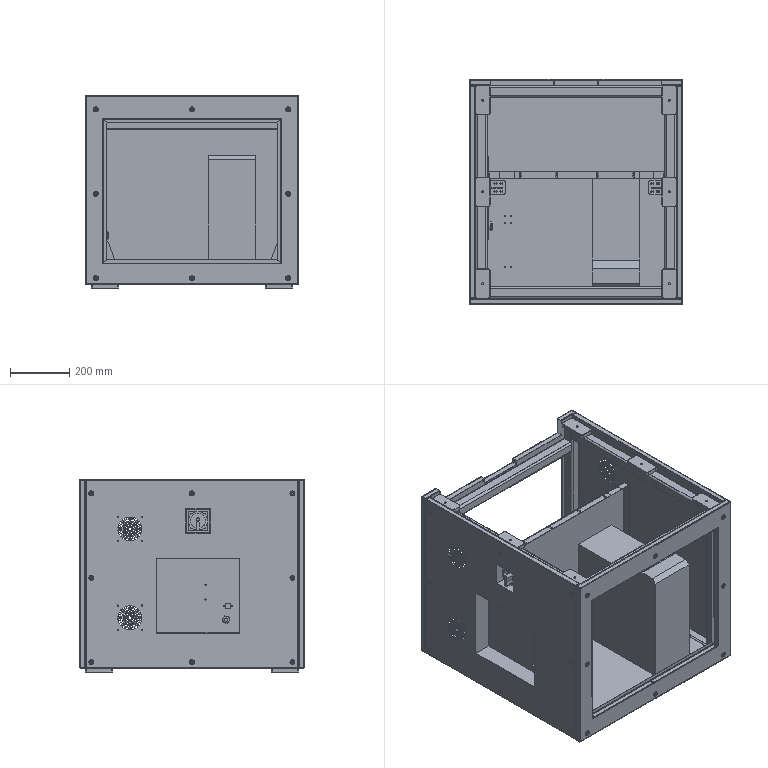Assembly | SolidWorks | mm | 22 component files | 35 solids | 2904 faces | box 720 x 760 x 652 mm | volume 31247087 mm3 | cylinder 1368 | plane 937 | torus 267 | spline 220 | cone 112 | commonest cylinder face diameters 5 x412 6.5 x86 15 x62 12 x62 6 x60 14 x48 1.473 x47 6.8 x44
Bill of materials:
01FrameBody | 1 | 4040 Square Tube | Open rectangular box-shaped frame made of square-section members: four vertical corner posts joined by horizontal rails at top and bottom on all four sides.
02LowerRackSpacer | 6 | A3 Steel | Rectangular block or thick plate with rounded corners, chamfered top and bottom edges, and one round through-hole in the centre.
03IntegratedCasterMount | 4 | A3 Steel | Square thick plate with small chamfered corners, chamfered edges, and four through-holes near the corners.
04CounterweightPlate | 1 | A3 Steel | Thin flat square sheet with slightly cut corners and a scattered pattern of small holes, some in four-hole groups and some single.
01-06LeftGuardPlate | 1 | SPCC | Flat rectangular panel with two round vent patterns, each made of concentric arc slots with a central hole and four small holes around it, plus eight holes spaced around the edge.
01-07RightGuardPlate | 1 | SPCC | Rectangular panel similar to a perforated plate, with two round slotted vent patterns, eight edge holes, and two raised rectangular box-shaped blocks on one face. It also has a small square cutout, a round hole and several small holes.
01-10ElectricalControlPanel | 1 | SGLCC | Shallow rectangular tray or pan: a flat panel with folded-up edges on all four sides. The longer flanges have elongated slots and the shorter flanges have round holes.
01-11FrontGuardPlate | 1 | SPCC | Flat rectangular frame with a large rectangular window that has a bevelled or stepped inner edge. The top edge has a tab rising at each end and a shallow notch in the middle. There are seven holes around the frame.
01-12RearGuardPlate | 1 | SPCC | Flat rectangular frame with a large rectangular window that has a bevelled or recessed inner edge, and eight holes evenly placed around the border.
01-16ElectricalControlPanelBracket | 1 | SGLCC | L-shaped bracket: a tall tapered vertical plate with three holes along one edge, a horizontal base flange with four elongated slots and rounded corners, and a triangular gusset between the two.
CableGlandPG13.5Black | 1 |  | Round hollow fitting with a domed end, a hexagonal nut section, a grooved neck, a larger hexagonal collar, and a grooved or ridged tube end. A round bore runs all the way through.
Host | 1 | Domestic 6061 | Solid rectangular block with a stepped, chamfered raised strip at one end of its top face, so one side profile has a small raised lip with angled edges.
Mirror01-16ElectricalControlPanelBracket | 1 | SUS304 | L-shaped plate bracket: a tall vertical web with one straight edge and one tapered edge, joined at a right angle to a short base flange that has four slotted holes. A triangular gusset plate runs between the flange and the web.
PowerSwitchTDS25-FRR | 1 |  | Flanged cylindrical body: a square plate with rounded corners and four corner holes, a short cylindrical shaft sticking out from the front face, a larger round disc-shaped body behind the plate, and a further protrusion on the rear.
Mates:
1. coincident | 01-01FrameBody-1/03IntegratedCasterMount-1 face at (0, 0, 0) dir (0, 0, -1) | assembly plane at (0, 0, 0) dir (0, 0, 1)
2. coincident | 01-01FrameBody-1/03IntegratedCasterMount-1 face at (-92, 0, 0) dir (0, -1, 0) | assembly plane at (0, 0, 0) dir (0, 1, 0)
3. coincident | 01-01FrameBody-1/03IntegratedCasterMount-1 face at (0, 92, 0) dir (1, 0, 0) | assembly plane at (0, 0, 0) dir (1, 0, 0)
4. coincident | 01-01FrameBody-1/01FrameBody-2 face at (-7, 720, 35) dir (0, 1, 0) | 01-11FrontGuardPlate-1 face at (6, 720, 17.207) dir (0, -1, 0)
5. coincident | 01-01FrameBody-1/01FrameBody-2 face at (-20, 687, 15) dir (0, 0, -1) | 01-11FrontGuardPlate-1 face at (-700, 720, 15) dir (0, 0, -1)
6. width | 01-11FrontGuardPlate-1 face at (20, 720, 15) dir (1, 0, 0) | 01-11FrontGuardPlate-1 face at (-700, 738.5, 15) dir (-1, 0, 0) | 01-01FrameBody-1/01FrameBody-2 face at (-680, 687, 35) dir (-1, 0, 0) | 01-01FrameBody-1/01FrameBody-2 face at (0, 687, 35) dir (1, 0, 0)
7. coincident | 01-01FrameBody-1/01FrameBody-2 face at (-20, 0, 618) dir (0, -1, 0) | 01-12RearGuardPlate-1 face at (17.793, 0, 650.5) dir (0, 1, 0)
8. coincident | 01-11FrontGuardPlate-1 face at (-700, 738.5, 15) dir (-1, 0, 0) | 01-12RearGuardPlate-1 face at (-700, 0, 15) dir (-1, 0, 0)
9. coincident | 01-11FrontGuardPlate-1 face at (20, 720, 652) dir (0, 0, 1) | 01-12RearGuardPlate-1 face at (-700, 0, 652) dir (0, 0, 1)
10. coincident | 01-01FrameBody-1/01FrameBody-2 face at (0, 20, 592) dir (1, 0, 0) | 01-06LeftGuardPlate-1 face at (0, 2.707, 638) dir (-1, 0, 0)
11. width | 01-06LeftGuardPlate-1 face at (0, 0.5, 15) dir (0, -1, 0) | 01-06LeftGuardPlate-1 face at (18.5, 719.5, 15) dir (0, 1, 0) | 01-11FrontGuardPlate-1 face at (20, 740, 652) dir (0, 1, 0) | 01-12RearGuardPlate-1 face at (-700, -20, 652) dir (0, -1, 0)
12. coincident | 01-06LeftGuardPlate-1 face at (0, 0.5, 652) dir (0, 0, 1) | 01-12RearGuardPlate-1 face at (-700, 0, 652) dir (0, 0, 1)
13. coincident | 01-01FrameBody-1/01FrameBody-2 face at (-680, 20, 592) dir (-1, 0, 0) | 01-07RightGuardPlate-1 face at (-680, 717.293, 638) dir (1, 0, 0)
14. coincident | 01-07RightGuardPlate-1 face at (-680, 719.5, 652) dir (0, 0, 1) | 01-12RearGuardPlate-1 face at (-700, 0, 652) dir (0, 0, 1)
15. width | 01-07RightGuardPlate-1 face at (-680, 719.5, 15) dir (0, 1, 0) | 01-07RightGuardPlate-1 face at (-698.5, 0.5, 15) dir (0, -1, 0) | 01-12RearGuardPlate-1 face at (-700, -20, 652) dir (0, -1, 0) | 01-11FrontGuardPlate-1 face at (20, 740, 652) dir (0, 1, 0)
16. coincident | 01-01FrameBody-1/04CounterweightPlate-4 face at (-640, 680, 55) dir (0, 0, 1) | 01-10ElectricalControlPanel-1 face at (-632, 405, 55) dir (0, 0, -1)
17. distance | 01-01FrameBody-1/01FrameBody-2 face at (0, 20, 22) dir (1, 0, 0) | 01-10ElectricalControlPanel-1 face at (-40, 405, 57) dir (1, 0, 0)
18. distance | 01-10ElectricalControlPanel-1 face at (-632, 430, 57) dir (0, 1, 0) | 01-01FrameBody-1/01FrameBody-2 face at (-20, 680, 48) dir (0, -1, 0)
19. coincident | 01-01FrameBody-1/04CounterweightPlate-4 face at (-640, 680, 55) dir (0, 0, 1) | Host-1 face at (-124.631, 35, 55) dir (0, 0, -1)
20. coincident | 01-01FrameBody-1/04CounterweightPlate-4 face at (-640, 680, 55) dir (0, 0, 1) | 01-16ElectricalControlPanelBracket-1 face at (-629, 353, 55) dir (0, 0, -1)
21. coincident | 01-10ElectricalControlPanel-1 face at (-632, 405, 537) dir (1, 0, 0) | 01-16ElectricalControlPanelBracket-1 face at (-632, 353, 258) dir (-1, 0, 0)
22. distance | 01-10ElectricalControlPanel-1 face at (-632, 428, 57) dir (0, -1, 0) | 01-16ElectricalControlPanelBracket-1 face at (-628.263, 418, 55) dir (0, 1, 0)
23. coincident | 01-10ElectricalControlPanel-1 face at (-632, 405, 55) dir (0, -1, 0) | Host-1 face at (-284.631, 405, 415) dir (0, 1, 0)
24. coincident | 01-07RightGuardPlate-1 face at (-660, 360, 333.5) dir (-1, 0, 0) | PowerSwitchTDS25-FRR-1 face at (-660, 372, 479.5) dir (1, 0, 0)
25. width | 01-07RightGuardPlate-1 face at (-658.5, 299.5, 333.5) dir (0, 1, 0) | 01-07RightGuardPlate-1 face at (-658.5, 379.5, 333.5) dir (0, -1, 0) | PowerSwitchTDS25-FRR-1 face at (-667, 307, 544.5) dir (0, -1, 0) | PowerSwitchTDS25-FRR-1 face at (-667, 372, 544.5) dir (0, 1, 0)
26. width | 01-07RightGuardPlate-1 face at (-658.5, 360, 552) dir (0, 0, -1) | 01-07RightGuardPlate-1 face at (-658.5, 360, 472) dir (0, 0, 1) | PowerSwitchTDS25-FRR-1 face at (-667, 372, 544.5) dir (0, 0, 1) | PowerSwitchTDS25-FRR-1 face at (-667, 372, 479.5) dir (0, 0, -1)
27. coincident | 01-07RightGuardPlate-1 face at (-638.5, 480, 383.5) dir (-1, 0, 0) | CableGlandPG13.5Black-1 face at (-638.5, 258.069, 180.851) dir (1, 0, 0)
28. concentric | 01-07RightGuardPlate-1 face at (-637, 245, 178.5) dir (-1, 0, 0) r 11.25 | CableGlandPG13.5Black-1 face at (-621.473, 245, 178.5) dir (-1, 0, 0) r 5.5
29. coincident | 03IntegratedCasterMount-2 face at (260.665, -242.877, -292.639) dir (0, 0, 1) | 01FrameBody-2 face at (260.665, -314.877, -292.639) dir (0, 0, -1)
30. coincident | 01FrameBody-2 face at (260.665, -327.877, -272.639) dir (1, 0, 0) | 03IntegratedCasterMount-2 face at (260.665, -334.877, -307.639) dir (1, 0, 0)
31. coincident | 01FrameBody-2 face at (227.665, -334.877, -272.639) dir (0, -1, 0) | 03IntegratedCasterMount-2 face at (168.665, -334.877, -307.639) dir (0, -1, 0)
32. coincident | 01FrameBody-2 face at (220.665, 325.123, -292.639) dir (0, 0, -1) | 03IntegratedCasterMount-3 face at (260.665, 345.123, -292.639) dir (0, 0, 1)
33. coincident | 01FrameBody-2 face at (227.665, 345.123, -272.639) dir (0, 1, 0) | 03IntegratedCasterMount-3 face at (168.665, 345.123, -307.639) dir (0, 1, 0)
34. coincident | 01FrameBody-2 face at (260.665, 312.123, -272.639) dir (1, 0, 0) | 03IntegratedCasterMount-3 face at (260.665, 253.123, -307.639) dir (1, 0, 0)
35. coincident | 01FrameBody-2 face at (-459.335, 325.123, -292.639) dir (0, 0, -1) | 03IntegratedCasterMount-4 face at (-367.335, 345.123, -292.639) dir (0, 0, 1)
36. coincident | 01FrameBody-2 face at (-452.335, 345.123, -272.639) dir (0, 1, 0) | 03IntegratedCasterMount-4 face at (-459.335, 345.123, -307.639) dir (0, 1, 0)
37. coincident | 01FrameBody-2 face at (-459.335, 312.123, -272.639) dir (-1, 0, 0) | 03IntegratedCasterMount-4 face at (-459.335, 253.123, -307.639) dir (-1, 0, 0)
38. coincident | 01FrameBody-2 face at (-419.335, -314.877, -292.639) dir (0, 0, -1) | 03IntegratedCasterMount-1 face at (-459.335, -334.877, -292.639) dir (0, 0, 1)
39. coincident | 01FrameBody-2 face at (-459.335, -327.877, -272.639) dir (-1, 0, 0) | 03IntegratedCasterMount-1 face at (-459.335, -242.877, -307.639) dir (-1, 0, 0)
40. coincident | 01FrameBody-2 face at (-452.335, -334.877, -272.639) dir (0, -1, 0) | 03IntegratedCasterMount-1 face at (-367.335, -334.877, -307.639) dir (0, -1, 0)
41. coincident | 01FrameBody-2 face at (-459.335, -314.877, 317.361) dir (0, 0, 1) | 02LowerRackSpacer-1 face at (-359.335, -334.877, 317.361) dir (0, 0, -1)
42. coincident | 01FrameBody-2 face at (-419.335, 325.123, 317.361) dir (0, 0, 1) | 02LowerRackSpacer-2 face at (-359.335, 345.123, 317.361) dir (0, 0, -1)
43. coincident | 01FrameBody-2 face at (240.665, 305.123, 317.361) dir (0, 0, 1) | 02LowerRackSpacer-6 face at (260.665, 295.123, 317.361) dir (0, 0, -1)
44. coincident | 01FrameBody-2 face at (260.665, 312.123, -272.639) dir (1, 0, 0) | 02LowerRackSpacer-6 face at (260.665, 345.123, 317.361) dir (1, 0, 0)
45. coincident | 01FrameBody-2 face at (227.665, 345.123, -272.639) dir (0, 1, 0) | 02LowerRackSpacer-6 face at (160.665, 345.123, 317.361) dir (0, 1, 0)
46. coincident | 01FrameBody-2 face at (240.665, -334.877, 317.361) dir (0, 0, 1) | 02LowerRackSpacer-5 face at (260.665, -334.877, 317.361) dir (0, 0, -1)
47. coincident | 01FrameBody-2 face at (227.665, -334.877, -272.639) dir (0, -1, 0) | 02LowerRackSpacer-5 face at (160.665, -334.877, 317.361) dir (0, -1, 0)
48. coincident | 01FrameBody-2 face at (260.665, -327.877, -272.639) dir (1, 0, 0) | 02LowerRackSpacer-5 face at (260.665, -284.877, 317.361) dir (1, 0, 0)
49. coincident | 01FrameBody-2 face at (-459.335, -327.877, -272.639) dir (-1, 0, 0) | 02LowerRackSpacer-1 face at (-459.335, -284.877, 317.361) dir (-1, 0, 0)
50. coincident | 01FrameBody-2 face at (-452.335, -334.877, -272.639) dir (0, -1, 0) | 02LowerRackSpacer-1 face at (-459.335, -334.877, 317.361) dir (0, -1, 0)
51. coincident | 01FrameBody-2 face at (-459.335, 312.123, -272.639) dir (-1, 0, 0) | 02LowerRackSpacer-2 face at (-459.335, 295.123, 332.361) dir (-1, 0, 0)
52. coincident | 01FrameBody-2 face at (-452.335, 345.123, -272.639) dir (0, 1, 0) | 02LowerRackSpacer-2 face at (-459.335, 345.123, 332.361) dir (0, 1, 0)
53. width | 04CounterweightPlate-4 face at (-419.335, -294.877, -252.639) dir (-1, 0, 0) | 04CounterweightPlate-4 face at (220.665, -294.877, -252.639) dir (1, 0, 0) | 01FrameBody-2 face at (260.665, -314.877, -259.639) dir (1, 0, 0) | 01FrameBody-2 face at (-459.335, -314.877, -259.639) dir (-1, 0, 0)
54. width | 04CounterweightPlate-4 face at (-419.335, -294.877, -252.639) dir (0, -1, 0) | 04CounterweightPlate-4 face at (-419.335, 305.123, -252.639) dir (0, 1, 0) | 01FrameBody-2 face at (-439.335, 345.123, -285.639) dir (0, 1, 0) | 01FrameBody-2 face at (-439.335, -334.877, -285.639) dir (0, -1, 0)
55. coincident | 01FrameBody-2 face at (-439.335, 338.123, -252.639) dir (0, 0, 1) | 04CounterweightPlate-4 face at (220.665, 305.123, -252.639) dir (0, 0, 1)
56. coincident | 01FrameBody-2 face at (-439.335, -301.877, 317.361) dir (0, 0, 1) | 02LowerRackSpacer-7 face at (-49.335, -334.877, 317.361) dir (0, 0, -1)
57. coincident | 02LowerRackSpacer-1 face at (-459.335, -334.877, 317.361) dir (0, -1, 0) | 02LowerRackSpacer-7 face at (-149.335, -334.877, 317.361) dir (0, -1, 0)
58. width | 02LowerRackSpacer-1 face at (-359.335, -284.877, 317.361) dir (1, 0, 0) | 02LowerRackSpacer-5 face at (160.665, -284.877, 317.361) dir (-1, 0, 0) | 02LowerRackSpacer-7 face at (-149.335, -284.877, 317.361) dir (-1, 0, 0) | 02LowerRackSpacer-7 face at (-49.335, -284.877, 317.361) dir (1, 0, 0)
59. coincident | 01FrameBody-2 face at (-439.335, 338.123, 317.361) dir (0, 0, 1) | 02LowerRackSpacer-8 face at (-49.335, 295.123, 317.361) dir (0, 0, -1)
60. coincident | 01FrameBody-2 face at (-439.335, 345.123, 284.361) dir (0, 1, 0) | 02LowerRackSpacer-8 face at (-149.335, 345.123, 317.361) dir (0, 1, 0)
61. width | 02LowerRackSpacer-2 face at (-359.335, 295.123, 332.361) dir (1, 0, 0) | 02LowerRackSpacer-6 face at (160.665, 345.123, 317.361) dir (-1, 0, 0) | 02LowerRackSpacer-8 face at (-149.335, 345.123, 317.361) dir (-1, 0, 0) | 02LowerRackSpacer-8 face at (-49.335, 345.123, 317.361) dir (1, 0, 0)